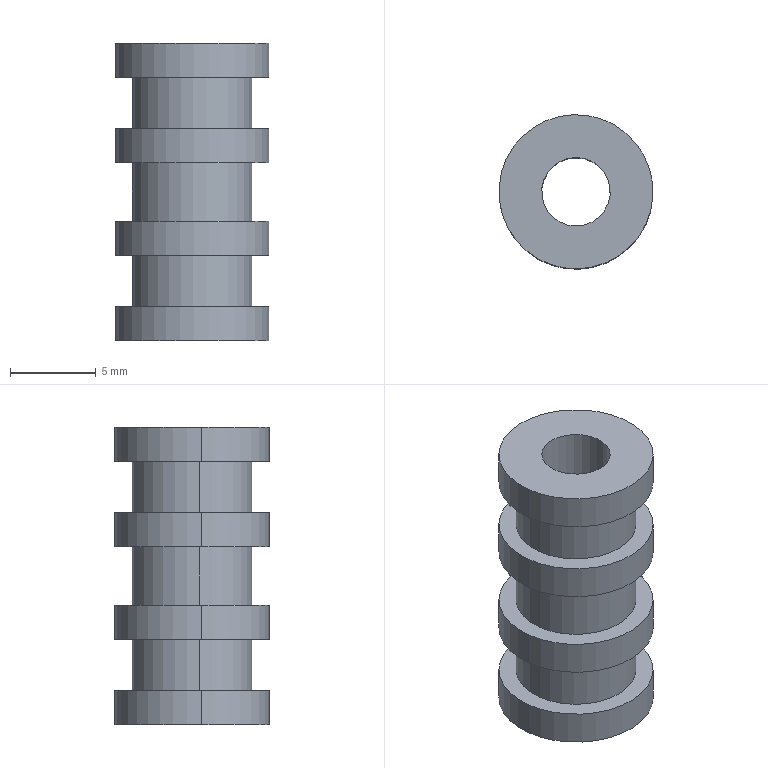Component | SolidWorks | TapeGuideRoller-1 | 1 solid | 24 faces | box 9 x 9 x 17.4 mm | volume 652 mm3 | cylinder 16 | plane 8 | commonest cylinder face diameters 9 x8 7 x6 4 x2
STEP:
#1=COLOUR_RGB('',0.7922,0.8196,0.9333);
#2=FILL_AREA_STYLE_COLOUR('',#1);
#3=FILL_AREA_STYLE('',(#2));
#4=SURFACE_STYLE_FILL_AREA(#3);
#5=SURFACE_SIDE_STYLE('',(#4));
#6=SURFACE_STYLE_USAGE(.BOTH.,#5);
#7=PRESENTATION_STYLE_ASSIGNMENT((#6));
#8=CARTESIAN_POINT('',(-6.397,4.985,1.713));
#9=VERTEX_POINT('',#8);
#10=CARTESIAN_POINT('',(-6.241,5.004,1.713));
#11=VERTEX_POINT('',#10);
#12=CARTESIAN_POINT('',(-6.319,4.995,1.713));
#13=DIRECTION('',(-0.,0.,-1.));
#14=DIRECTION('',(0.9922,0.1244,0.));
#15=AXIS2_PLACEMENT_3D('',#12,#13,#14);
#16=CIRCLE('',#15,0.07874);
#17=EDGE_CURVE('',#9,#11,#16,.T.);
#18=ORIENTED_EDGE('',*,*,#17,.F.);
#19=CARTESIAN_POINT('',(-6.397,4.985,1.028));
#20=VERTEX_POINT('',#19);
#21=CARTESIAN_POINT('',(-6.397,4.985,0.4858));
#22=DIRECTION('',(-0.,0.,-1.));
#23=VECTOR('',#22,39.37);
#24=LINE('',#21,#23);
#25=EDGE_CURVE('',#9,#20,#24,.T.);
#26=ORIENTED_EDGE('',*,*,#25,.T.);
#27=CARTESIAN_POINT('',(-6.241,5.004,1.028));
#28=VERTEX_POINT('',#27);
#29=CARTESIAN_POINT('',(-6.319,4.995,1.028));
#30=DIRECTION('',(0.,-0.,1.));
#31=DIRECTION('',(0.9922,0.1244,0.));
#32=AXIS2_PLACEMENT_3D('',#29,#30,#31);
#33=CIRCLE('',#32,0.07874);
#34=EDGE_CURVE('',#28,#20,#33,.T.);
#35=ORIENTED_EDGE('',*,*,#34,.F.);
#36=CARTESIAN_POINT('',(-6.241,5.004,0.4858));
#37=DIRECTION('',(-0.,0.,-1.));
#38=VECTOR('',#37,39.37);
#39=LINE('',#36,#38);
#40=EDGE_CURVE('',#11,#28,#39,.T.);
#41=ORIENTED_EDGE('',*,*,#40,.F.);
#42=EDGE_LOOP('',(#18,#26,#35,#41));
#43=FACE_OUTER_BOUND('',#42,.T.);
#44=CARTESIAN_POINT('',(-6.319,4.995,0.4858));
#45=DIRECTION('',(-0.,0.,-1.));
#46=DIRECTION('',(0.9922,0.1244,0.));
#47=AXIS2_PLACEMENT_3D('',#44,#45,#46);
#48=CYLINDRICAL_SURFACE('',#47,0.07874);
#49=ADVANCED_FACE('',(#43),#48,.F.);
#50=CARTESIAN_POINT('',(-6.143,5.017,1.713));
#51=VERTEX_POINT('',#50);
#52=CARTESIAN_POINT('',(-6.495,4.973,1.713));
#53=VERTEX_POINT('',#52);
#54=CARTESIAN_POINT('',(-6.319,4.995,1.713));
#55=DIRECTION('',(-0.,0.,-1.));
#56=DIRECTION('',(0.9922,0.1244,0.));
#57=AXIS2_PLACEMENT_3D('',#54,#55,#56);
#58=CIRCLE('',#57,0.1772);
#59=EDGE_CURVE('',#51,#53,#58,.T.);
#60=ORIENTED_EDGE('',*,*,#59,.T.);
#61=CARTESIAN_POINT('',(-6.495,4.973,1.634));
#62=VERTEX_POINT('',#61);
#63=CARTESIAN_POINT('',(-6.495,4.973,0.4858));
#64=DIRECTION('',(-0.,0.,-1.));
#65=VECTOR('',#64,39.37);
#66=LINE('',#63,#65);
#67=EDGE_CURVE('',#53,#62,#66,.T.);
#68=ORIENTED_EDGE('',*,*,#67,.T.);
#69=CARTESIAN_POINT('',(-6.143,5.017,1.634));
#70=VERTEX_POINT('',#69);
#71=CARTESIAN_POINT('',(-6.319,4.995,1.634));
#72=DIRECTION('',(0.,-0.,1.));
#73=DIRECTION('',(0.9922,0.1244,0.));
#74=AXIS2_PLACEMENT_3D('',#71,#72,#73);
#75=CIRCLE('',#74,0.1772);
#76=EDGE_CURVE('',#62,#70,#75,.T.);
#77=ORIENTED_EDGE('',*,*,#76,.T.);
#78=CARTESIAN_POINT('',(-6.143,5.017,0.4858));
#79=DIRECTION('',(-0.,0.,-1.));
#80=VECTOR('',#79,39.37);
#81=LINE('',#78,#80);
#82=EDGE_CURVE('',#51,#70,#81,.T.);
#83=ORIENTED_EDGE('',*,*,#82,.F.);
#84=EDGE_LOOP('',(#60,#68,#77,#83));
#85=FACE_OUTER_BOUND('',#84,.T.);
#86=CARTESIAN_POINT('',(-6.319,4.995,0.4858));
#87=DIRECTION('',(-0.,0.,-1.));
#88=DIRECTION('',(0.9922,0.1244,0.));
#89=AXIS2_PLACEMENT_3D('',#86,#87,#88);
#90=CYLINDRICAL_SURFACE('',#89,0.1772);
#91=ADVANCED_FACE('',(#85),#90,.T.);
#92=CARTESIAN_POINT('',(-6.143,5.017,1.106));
#93=VERTEX_POINT('',#92);
#94=CARTESIAN_POINT('',(-6.495,4.973,1.106));
#95=VERTEX_POINT('',#94);
#96=CARTESIAN_POINT('',(-6.319,4.995,1.106));
#97=DIRECTION('',(-0.,0.,-1.));
#98=DIRECTION('',(0.9922,0.1244,0.));
#99=AXIS2_PLACEMENT_3D('',#96,#97,#98);
#100=CIRCLE('',#99,0.1772);
#101=EDGE_CURVE('',#93,#95,#100,.T.);
#102=ORIENTED_EDGE('',*,*,#101,.T.);
#103=CARTESIAN_POINT('',(-6.495,4.973,1.028));
#104=VERTEX_POINT('',#103);
#105=CARTESIAN_POINT('',(-6.495,4.973,0.4858));
#106=DIRECTION('',(-0.,0.,-1.));
#107=VECTOR('',#106,39.37);
#108=LINE('',#105,#107);
#109=EDGE_CURVE('',#95,#104,#108,.T.);
#110=ORIENTED_EDGE('',*,*,#109,.T.);
#111=CARTESIAN_POINT('',(-6.143,5.017,1.028));
#112=VERTEX_POINT('',#111);
#113=CARTESIAN_POINT('',(-6.319,4.995,1.028));
#114=DIRECTION('',(0.,-0.,1.));
#115=DIRECTION('',(0.9922,0.1244,0.));
#116=AXIS2_PLACEMENT_3D('',#113,#114,#115);
#117=CIRCLE('',#116,0.1772);
#118=EDGE_CURVE('',#104,#112,#117,.T.);
#119=ORIENTED_EDGE('',*,*,#118,.T.);
#120=CARTESIAN_POINT('',(-6.143,5.017,0.4858));
#121=DIRECTION('',(-0.,0.,-1.));
#122=VECTOR('',#121,39.37);
#123=LINE('',#120,#122);
#124=EDGE_CURVE('',#93,#112,#123,.T.);
#125=ORIENTED_EDGE('',*,*,#124,.F.);
#126=EDGE_LOOP('',(#102,#110,#119,#125));
#127=FACE_OUTER_BOUND('',#126,.T.);
#128=CARTESIAN_POINT('',(-6.319,4.995,0.4858));
#129=DIRECTION('',(-0.,0.,-1.));
#130=DIRECTION('',(0.9922,0.1244,0.));
#131=AXIS2_PLACEMENT_3D('',#128,#129,#130);
#132=CYLINDRICAL_SURFACE('',#131,0.1772);
#133=ADVANCED_FACE('',(#127),#132,.T.);
#134=CARTESIAN_POINT('',(-6.182,5.012,1.634));
#135=VERTEX_POINT('',#134);
#136=CARTESIAN_POINT('',(-6.456,4.978,1.634));
#137=VERTEX_POINT('',#136);
#138=CARTESIAN_POINT('',(-6.319,4.995,1.634));
#139=DIRECTION('',(-0.,0.,-1.));
#140=DIRECTION('',(0.9922,0.1244,0.));
#141=AXIS2_PLACEMENT_3D('',#138,#139,#140);
#142=CIRCLE('',#141,0.1378);
#143=EDGE_CURVE('',#135,#137,#142,.T.);
#144=ORIENTED_EDGE('',*,*,#143,.T.);
#145=CARTESIAN_POINT('',(-6.456,4.978,1.516));
#146=VERTEX_POINT('',#145);
#147=CARTESIAN_POINT('',(-6.456,4.978,0.4858));
#148=DIRECTION('',(-0.,0.,-1.));
#149=VECTOR('',#148,39.37);
#150=LINE('',#147,#149);
#151=EDGE_CURVE('',#137,#146,#150,.T.);
#152=ORIENTED_EDGE('',*,*,#151,.T.);
#153=CARTESIAN_POINT('',(-6.182,5.012,1.516));
#154=VERTEX_POINT('',#153);
#155=CARTESIAN_POINT('',(-6.319,4.995,1.516));
#156=DIRECTION('',(0.,-0.,1.));
#157=DIRECTION('',(0.9922,0.1244,0.));
#158=AXIS2_PLACEMENT_3D('',#155,#156,#157);
#159=CIRCLE('',#158,0.1378);
#160=EDGE_CURVE('',#146,#154,#159,.T.);
#161=ORIENTED_EDGE('',*,*,#160,.T.);
#162=CARTESIAN_POINT('',(-6.182,5.012,0.4858));
#163=DIRECTION('',(-0.,0.,-1.));
#164=VECTOR('',#163,39.37);
#165=LINE('',#162,#164);
#166=EDGE_CURVE('',#135,#154,#165,.T.);
#167=ORIENTED_EDGE('',*,*,#166,.F.);
#168=EDGE_LOOP('',(#144,#152,#161,#167));
#169=FACE_OUTER_BOUND('',#168,.T.);
#170=CARTESIAN_POINT('',(-6.319,4.995,0.4858));
#171=DIRECTION('',(-0.,0.,-1.));
#172=DIRECTION('',(0.9922,0.1244,0.));
#173=AXIS2_PLACEMENT_3D('',#170,#171,#172);
#174=CYLINDRICAL_SURFACE('',#173,0.1378);
#175=ADVANCED_FACE('',(#169),#174,.T.);
#176=CARTESIAN_POINT('',(-6.182,5.012,1.224));
#177=VERTEX_POINT('',#176);
#178=CARTESIAN_POINT('',(-6.456,4.978,1.224));
#179=VERTEX_POINT('',#178);
#180=CARTESIAN_POINT('',(-6.319,4.995,1.224));
#181=DIRECTION('',(-0.,0.,-1.));
#182=DIRECTION('',(0.9922,0.1244,0.));
#183=AXIS2_PLACEMENT_3D('',#180,#181,#182);
#184=CIRCLE('',#183,0.1378);
#185=EDGE_CURVE('',#177,#179,#184,.T.);
#186=ORIENTED_EDGE('',*,*,#185,.T.);
#187=CARTESIAN_POINT('',(-6.456,4.978,1.106));
#188=VERTEX_POINT('',#187);
#189=CARTESIAN_POINT('',(-6.456,4.978,0.4858));
#190=DIRECTION('',(-0.,0.,-1.));
#191=VECTOR('',#190,39.37);
#192=LINE('',#189,#191);
#193=EDGE_CURVE('',#179,#188,#192,.T.);
#194=ORIENTED_EDGE('',*,*,#193,.T.);
#195=CARTESIAN_POINT('',(-6.182,5.012,1.106));
#196=VERTEX_POINT('',#195);
#197=CARTESIAN_POINT('',(-6.319,4.995,1.106));
#198=DIRECTION('',(0.,-0.,1.));
#199=DIRECTION('',(0.9922,0.1244,0.));
#200=AXIS2_PLACEMENT_3D('',#197,#198,#199);
#201=CIRCLE('',#200,0.1378);
#202=EDGE_CURVE('',#188,#196,#201,.T.);
#203=ORIENTED_EDGE('',*,*,#202,.T.);
#204=CARTESIAN_POINT('',(-6.182,5.012,0.4858));
#205=DIRECTION('',(-0.,0.,-1.));
#206=VECTOR('',#205,39.37);
#207=LINE('',#204,#206);
#208=EDGE_CURVE('',#177,#196,#207,.T.);
#209=ORIENTED_EDGE('',*,*,#208,.F.);
#210=EDGE_LOOP('',(#186,#194,#203,#209));
#211=FACE_OUTER_BOUND('',#210,.T.);
#212=CARTESIAN_POINT('',(-6.319,4.995,0.4858));
#213=DIRECTION('',(-0.,0.,-1.));
#214=DIRECTION('',(0.9922,0.1244,0.));
#215=AXIS2_PLACEMENT_3D('',#212,#213,#214);
#216=CYLINDRICAL_SURFACE('',#215,0.1378);
#217=ADVANCED_FACE('',(#211),#216,.T.);
#218=CARTESIAN_POINT('',(-6.143,5.017,1.516));
#219=VERTEX_POINT('',#218);
#220=CARTESIAN_POINT('',(-6.495,4.973,1.516));
#221=VERTEX_POINT('',#220);
#222=CARTESIAN_POINT('',(-6.319,4.995,1.516));
#223=DIRECTION('',(-0.,0.,-1.));
#224=DIRECTION('',(0.9922,0.1244,0.));
#225=AXIS2_PLACEMENT_3D('',#222,#223,#224);
#226=CIRCLE('',#225,0.1772);
#227=EDGE_CURVE('',#219,#221,#226,.T.);
#228=ORIENTED_EDGE('',*,*,#227,.T.);
#229=CARTESIAN_POINT('',(-6.495,4.973,1.437));
#230=VERTEX_POINT('',#229);
#231=CARTESIAN_POINT('',(-6.495,4.973,0.4858));
#232=DIRECTION('',(-0.,0.,-1.));
#233=VECTOR('',#232,39.37);
#234=LINE('',#231,#233);
#235=EDGE_CURVE('',#221,#230,#234,.T.);
#236=ORIENTED_EDGE('',*,*,#235,.T.);
#237=CARTESIAN_POINT('',(-6.143,5.017,1.437));
#238=VERTEX_POINT('',#237);
#239=CARTESIAN_POINT('',(-6.319,4.995,1.437));
#240=DIRECTION('',(0.,-0.,1.));
#241=DIRECTION('',(0.9922,0.1244,0.));
#242=AXIS2_PLACEMENT_3D('',#239,#240,#241);
#243=CIRCLE('',#242,0.1772);
#244=EDGE_CURVE('',#230,#238,#243,.T.);
#245=ORIENTED_EDGE('',*,*,#244,.T.);
#246=CARTESIAN_POINT('',(-6.143,5.017,0.4858));
#247=DIRECTION('',(-0.,0.,-1.));
#248=VECTOR('',#247,39.37);
#249=LINE('',#246,#248);
#250=EDGE_CURVE('',#219,#238,#249,.T.);
#251=ORIENTED_EDGE('',*,*,#250,.F.);
#252=EDGE_LOOP('',(#228,#236,#245,#251));
#253=FACE_OUTER_BOUND('',#252,.T.);
#254=CARTESIAN_POINT('',(-6.319,4.995,0.4858));
#255=DIRECTION('',(-0.,0.,-1.));
#256=DIRECTION('',(0.9922,0.1244,0.));
#257=AXIS2_PLACEMENT_3D('',#254,#255,#256);
#258=CYLINDRICAL_SURFACE('',#257,0.1772);
#259=ADVANCED_FACE('',(#253),#258,.T.);
#260=CARTESIAN_POINT('',(-6.143,5.017,1.303));
#261=VERTEX_POINT('',#260);
#262=CARTESIAN_POINT('',(-6.495,4.973,1.303));
#263=VERTEX_POINT('',#262);
#264=CARTESIAN_POINT('',(-6.319,4.995,1.303));
#265=DIRECTION('',(-0.,0.,-1.));
#266=DIRECTION('',(0.9922,0.1244,0.));
#267=AXIS2_PLACEMENT_3D('',#264,#265,#266);
#268=CIRCLE('',#267,0.1772);
#269=EDGE_CURVE('',#261,#263,#268,.T.);
#270=ORIENTED_EDGE('',*,*,#269,.T.);
#271=CARTESIAN_POINT('',(-6.495,4.973,1.224));
#272=VERTEX_POINT('',#271);
#273=CARTESIAN_POINT('',(-6.495,4.973,0.4858));
#274=DIRECTION('',(-0.,0.,-1.));
#275=VECTOR('',#274,39.37);
#276=LINE('',#273,#275);
#277=EDGE_CURVE('',#263,#272,#276,.T.);
#278=ORIENTED_EDGE('',*,*,#277,.T.);
#279=CARTESIAN_POINT('',(-6.143,5.017,1.224));
#280=VERTEX_POINT('',#279);
#281=CARTESIAN_POINT('',(-6.319,4.995,1.224));
#282=DIRECTION('',(0.,-0.,1.));
#283=DIRECTION('',(0.9922,0.1244,0.));
#284=AXIS2_PLACEMENT_3D('',#281,#282,#283);
#285=CIRCLE('',#284,0.1772);
#286=EDGE_CURVE('',#272,#280,#285,.T.);
#287=ORIENTED_EDGE('',*,*,#286,.T.);
#288=CARTESIAN_POINT('',(-6.143,5.017,0.4858));
#289=DIRECTION('',(-0.,0.,-1.));
#290=VECTOR('',#289,39.37);
#291=LINE('',#288,#290);
#292=EDGE_CURVE('',#261,#280,#291,.T.);
#293=ORIENTED_EDGE('',*,*,#292,.F.);
#294=EDGE_LOOP('',(#270,#278,#287,#293));
#295=FACE_OUTER_BOUND('',#294,.T.);
#296=CARTESIAN_POINT('',(-6.319,4.995,0.4858));
#297=DIRECTION('',(-0.,0.,-1.));
#298=DIRECTION('',(0.9922,0.1244,0.));
#299=AXIS2_PLACEMENT_3D('',#296,#297,#298);
#300=CYLINDRICAL_SURFACE('',#299,0.1772);
#301=ADVANCED_FACE('',(#295),#300,.T.);
#302=CARTESIAN_POINT('',(-6.182,5.012,1.437));
#303=VERTEX_POINT('',#302);
#304=CARTESIAN_POINT('',(-6.456,4.978,1.437));
#305=VERTEX_POINT('',#304);
#306=CARTESIAN_POINT('',(-6.319,4.995,1.437));
#307=DIRECTION('',(-0.,0.,-1.));
#308=DIRECTION('',(0.9922,0.1244,0.));
#309=AXIS2_PLACEMENT_3D('',#306,#307,#308);
#310=CIRCLE('',#309,0.1378);
#311=EDGE_CURVE('',#303,#305,#310,.T.);
#312=ORIENTED_EDGE('',*,*,#311,.T.);
#313=CARTESIAN_POINT('',(-6.456,4.978,1.303));
#314=VERTEX_POINT('',#313);
#315=CARTESIAN_POINT('',(-6.456,4.978,0.4858));
#316=DIRECTION('',(-0.,0.,-1.));
#317=VECTOR('',#316,39.37);
#318=LINE('',#315,#317);
#319=EDGE_CURVE('',#305,#314,#318,.T.);
#320=ORIENTED_EDGE('',*,*,#319,.T.);
#321=CARTESIAN_POINT('',(-6.182,5.012,1.303));
#322=VERTEX_POINT('',#321);
#323=CARTESIAN_POINT('',(-6.319,4.995,1.303));
#324=DIRECTION('',(0.,-0.,1.));
#325=DIRECTION('',(0.9922,0.1244,0.));
#326=AXIS2_PLACEMENT_3D('',#323,#324,#325);
#327=CIRCLE('',#326,0.1378);
#328=EDGE_CURVE('',#314,#322,#327,.T.);
#329=ORIENTED_EDGE('',*,*,#328,.T.);
#330=CARTESIAN_POINT('',(-6.182,5.012,0.4858));
#331=DIRECTION('',(-0.,0.,-1.));
#332=VECTOR('',#331,39.37);
#333=LINE('',#330,#332);
#334=EDGE_CURVE('',#303,#322,#333,.T.);
#335=ORIENTED_EDGE('',*,*,#334,.F.);
#336=EDGE_LOOP('',(#312,#320,#329,#335));
#337=FACE_OUTER_BOUND('',#336,.T.);
#338=CARTESIAN_POINT('',(-6.319,4.995,0.4858));
#339=DIRECTION('',(-0.,0.,-1.));
#340=DIRECTION('',(0.9922,0.1244,0.));
#341=AXIS2_PLACEMENT_3D('',#338,#339,#340);
#342=CYLINDRICAL_SURFACE('',#341,0.1378);
#343=ADVANCED_FACE('',(#337),#342,.T.);
#344=ORIENTED_EDGE('',*,*,#25,.F.);
#345=CARTESIAN_POINT('',(-6.319,4.995,1.713));
#346=DIRECTION('',(-0.,0.,-1.));
#347=DIRECTION('',(0.9922,0.1244,0.));
#348=AXIS2_PLACEMENT_3D('',#345,#346,#347);
#349=CIRCLE('',#348,0.07874);
#350=EDGE_CURVE('',#11,#9,#349,.T.);
#351=ORIENTED_EDGE('',*,*,#350,.F.);
#352=ORIENTED_EDGE('',*,*,#40,.T.);
#353=CARTESIAN_POINT('',(-6.319,4.995,1.028));
#354=DIRECTION('',(0.,-0.,1.));
#355=DIRECTION('',(0.9922,0.1244,0.));
#356=AXIS2_PLACEMENT_3D('',#353,#354,#355);
#357=CIRCLE('',#356,0.07874);
#358=EDGE_CURVE('',#20,#28,#357,.T.);
#359=ORIENTED_EDGE('',*,*,#358,.F.);
#360=EDGE_LOOP('',(#344,#351,#352,#359));
#361=FACE_OUTER_BOUND('',#360,.T.);
#362=CARTESIAN_POINT('',(-6.319,4.995,0.4858));
#363=DIRECTION('',(-0.,0.,-1.));
#364=DIRECTION('',(0.9922,0.1244,0.));
#365=AXIS2_PLACEMENT_3D('',#362,#363,#364);
#366=CYLINDRICAL_SURFACE('',#365,0.07874);
#367=ADVANCED_FACE('',(#361),#366,.F.);
#368=ORIENTED_EDGE('',*,*,#350,.T.);
#369=ORIENTED_EDGE('',*,*,#17,.T.);
#370=EDGE_LOOP('',(#368,#369));
#371=FACE_BOUND('',#370,.T.);
#372=ORIENTED_EDGE('',*,*,#59,.F.);
#373=CARTESIAN_POINT('',(-6.319,4.995,1.713));
#374=DIRECTION('',(-0.,0.,-1.));
#375=DIRECTION('',(0.9922,0.1244,0.));
#376=AXIS2_PLACEMENT_3D('',#373,#374,#375);
#377=CIRCLE('',#376,0.1772);
#378=EDGE_CURVE('',#53,#51,#377,.T.);
#379=ORIENTED_EDGE('',*,*,#378,.F.);
#380=EDGE_LOOP('',(#372,#379));
#381=FACE_OUTER_BOUND('',#380,.T.);
#382=CARTESIAN_POINT('',(-6.297,4.819,1.713));
#383=DIRECTION('',(-0.,0.,-1.));
#384=DIRECTION('',(0.9922,0.1244,0.));
#385=AXIS2_PLACEMENT_3D('',#382,#383,#384);
#386=PLANE('',#385);
#387=ADVANCED_FACE('',(#371,#381),#386,.F.);
#388=CARTESIAN_POINT('',(-6.319,4.995,1.028));
#389=DIRECTION('',(0.,-0.,1.));
#390=DIRECTION('',(0.9922,0.1244,0.));
#391=AXIS2_PLACEMENT_3D('',#388,#389,#390);
#392=CIRCLE('',#391,0.1772);
#393=EDGE_CURVE('',#112,#104,#392,.T.);
#394=ORIENTED_EDGE('',*,*,#393,.F.);
#395=ORIENTED_EDGE('',*,*,#118,.F.);
#396=EDGE_LOOP('',(#394,#395));
#397=FACE_OUTER_BOUND('',#396,.T.);
#398=ORIENTED_EDGE('',*,*,#34,.T.);
#399=ORIENTED_EDGE('',*,*,#358,.T.);
#400=EDGE_LOOP('',(#398,#399));
#401=FACE_BOUND('',#400,.T.);
#402=CARTESIAN_POINT('',(-6.297,4.819,1.028));
#403=DIRECTION('',(0.,-0.,1.));
#404=DIRECTION('',(-0.9922,-0.1244,-0.));
#405=AXIS2_PLACEMENT_3D('',#402,#403,#404);
#406=PLANE('',#405);
#407=ADVANCED_FACE('',(#397,#401),#406,.F.);
#408=ORIENTED_EDGE('',*,*,#67,.F.);
#409=ORIENTED_EDGE('',*,*,#378,.T.);
#410=ORIENTED_EDGE('',*,*,#82,.T.);
#411=CARTESIAN_POINT('',(-6.319,4.995,1.634));
#412=DIRECTION('',(0.,-0.,1.));
#413=DIRECTION('',(0.9922,0.1244,0.));
#414=AXIS2_PLACEMENT_3D('',#411,#412,#413);
#415=CIRCLE('',#414,0.1772);
#416=EDGE_CURVE('',#70,#62,#415,.T.);
#417=ORIENTED_EDGE('',*,*,#416,.T.);
#418=EDGE_LOOP('',(#408,#409,#410,#417));
#419=FACE_OUTER_BOUND('',#418,.T.);
#420=CARTESIAN_POINT('',(-6.319,4.995,0.4858));
#421=DIRECTION('',(-0.,0.,-1.));
#422=DIRECTION('',(0.9922,0.1244,0.));
#423=AXIS2_PLACEMENT_3D('',#420,#421,#422);
#424=CYLINDRICAL_SURFACE('',#423,0.1772);
#425=ADVANCED_FACE('',(#419),#424,.T.);
#426=ORIENTED_EDGE('',*,*,#109,.F.);
#427=CARTESIAN_POINT('',(-6.319,4.995,1.106));
#428=DIRECTION('',(-0.,0.,-1.));
#429=DIRECTION('',(0.9922,0.1244,0.));
#430=AXIS2_PLACEMENT_3D('',#427,#428,#429);
#431=CIRCLE('',#430,0.1772);
#432=EDGE_CURVE('',#95,#93,#431,.T.);
#433=ORIENTED_EDGE('',*,*,#432,.T.);
#434=ORIENTED_EDGE('',*,*,#124,.T.);
#435=ORIENTED_EDGE('',*,*,#393,.T.);
#436=EDGE_LOOP('',(#426,#433,#434,#435));
#437=FACE_OUTER_BOUND('',#436,.T.);
#438=CARTESIAN_POINT('',(-6.319,4.995,0.4858));
#439=DIRECTION('',(-0.,0.,-1.));
#440=DIRECTION('',(0.9922,0.1244,0.));
#441=AXIS2_PLACEMENT_3D('',#438,#439,#440);
#442=CYLINDRICAL_SURFACE('',#441,0.1772);
#443=ADVANCED_FACE('',(#437),#442,.T.);
#444=ORIENTED_EDGE('',*,*,#416,.F.);
#445=ORIENTED_EDGE('',*,*,#76,.F.);
#446=EDGE_LOOP('',(#444,#445));
#447=FACE_OUTER_BOUND('',#446,.T.);
#448=ORIENTED_EDGE('',*,*,#143,.F.);
#449=CARTESIAN_POINT('',(-6.319,4.995,1.634));
#450=DIRECTION('',(-0.,0.,-1.));
#451=DIRECTION('',(0.9922,0.1244,0.));
#452=AXIS2_PLACEMENT_3D('',#449,#450,#451);
#453=CIRCLE('',#452,0.1378);
#454=EDGE_CURVE('',#137,#135,#453,.T.);
#455=ORIENTED_EDGE('',*,*,#454,.F.);
#456=EDGE_LOOP('',(#448,#455));
#457=FACE_BOUND('',#456,.T.);
#458=CARTESIAN_POINT('',(-6.302,4.858,1.634));
#459=DIRECTION('',(0.,-0.,1.));
#460=DIRECTION('',(-0.9922,-0.1244,-0.));
#461=AXIS2_PLACEMENT_3D('',#458,#459,#460);
#462=PLANE('',#461);
#463=ADVANCED_FACE('',(#447,#457),#462,.F.);
#464=CARTESIAN_POINT('',(-6.319,4.995,1.106));
#465=DIRECTION('',(0.,-0.,1.));
#466=DIRECTION('',(0.9922,0.1244,0.));
#467=AXIS2_PLACEMENT_3D('',#464,#465,#466);
#468=CIRCLE('',#467,0.1378);
#469=EDGE_CURVE('',#196,#188,#468,.T.);
#470=ORIENTED_EDGE('',*,*,#469,.F.);
#471=ORIENTED_EDGE('',*,*,#202,.F.);
#472=EDGE_LOOP('',(#470,#471));
#473=FACE_BOUND('',#472,.T.);
#474=ORIENTED_EDGE('',*,*,#101,.F.);
#475=ORIENTED_EDGE('',*,*,#432,.F.);
#476=EDGE_LOOP('',(#474,#475));
#477=FACE_OUTER_BOUND('',#476,.T.);
#478=CARTESIAN_POINT('',(-6.297,4.819,1.106));
#479=DIRECTION('',(-0.,0.,-1.));
#480=DIRECTION('',(0.9922,0.1244,0.));
#481=AXIS2_PLACEMENT_3D('',#478,#479,#480);
#482=PLANE('',#481);
#483=ADVANCED_FACE('',(#473,#477),#482,.F.);
#484=ORIENTED_EDGE('',*,*,#151,.F.);
#485=ORIENTED_EDGE('',*,*,#454,.T.);
#486=ORIENTED_EDGE('',*,*,#166,.T.);
#487=CARTESIAN_POINT('',(-6.319,4.995,1.516));
#488=DIRECTION('',(0.,-0.,1.));
#489=DIRECTION('',(0.9922,0.1244,0.));
#490=AXIS2_PLACEMENT_3D('',#487,#488,#489);
#491=CIRCLE('',#490,0.1378);
#492=EDGE_CURVE('',#154,#146,#491,.T.);
#493=ORIENTED_EDGE('',*,*,#492,.T.);
#494=EDGE_LOOP('',(#484,#485,#486,#493));
#495=FACE_OUTER_BOUND('',#494,.T.);
#496=CARTESIAN_POINT('',(-6.319,4.995,0.4858));
#497=DIRECTION('',(-0.,0.,-1.));
#498=DIRECTION('',(0.9922,0.1244,0.));
#499=AXIS2_PLACEMENT_3D('',#496,#497,#498);
#500=CYLINDRICAL_SURFACE('',#499,0.1378);
#501=ADVANCED_FACE('',(#495),#500,.T.);
#502=ORIENTED_EDGE('',*,*,#193,.F.);
#503=CARTESIAN_POINT('',(-6.319,4.995,1.224));
#504=DIRECTION('',(-0.,0.,-1.));
#505=DIRECTION('',(0.9922,0.1244,0.));
#506=AXIS2_PLACEMENT_3D('',#503,#504,#505);
#507=CIRCLE('',#506,0.1378);
#508=EDGE_CURVE('',#179,#177,#507,.T.);
#509=ORIENTED_EDGE('',*,*,#508,.T.);
#510=ORIENTED_EDGE('',*,*,#208,.T.);
#511=ORIENTED_EDGE('',*,*,#469,.T.);
#512=EDGE_LOOP('',(#502,#509,#510,#511));
#513=FACE_OUTER_BOUND('',#512,.T.);
#514=CARTESIAN_POINT('',(-6.319,4.995,0.4858));
#515=DIRECTION('',(-0.,0.,-1.));
#516=DIRECTION('',(0.9922,0.1244,0.));
#517=AXIS2_PLACEMENT_3D('',#514,#515,#516);
#518=CYLINDRICAL_SURFACE('',#517,0.1378);
#519=ADVANCED_FACE('',(#513),#518,.T.);
#520=ORIENTED_EDGE('',*,*,#492,.F.);
#521=ORIENTED_EDGE('',*,*,#160,.F.);
#522=EDGE_LOOP('',(#520,#521));
#523=FACE_BOUND('',#522,.T.);
#524=ORIENTED_EDGE('',*,*,#227,.F.);
#525=CARTESIAN_POINT('',(-6.319,4.995,1.516));
#526=DIRECTION('',(-0.,0.,-1.));
#527=DIRECTION('',(0.9922,0.1244,0.));
#528=AXIS2_PLACEMENT_3D('',#525,#526,#527);
#529=CIRCLE('',#528,0.1772);
#530=EDGE_CURVE('',#221,#219,#529,.T.);
#531=ORIENTED_EDGE('',*,*,#530,.F.);
#532=EDGE_LOOP('',(#524,#531));
#533=FACE_OUTER_BOUND('',#532,.T.);
#534=CARTESIAN_POINT('',(-6.297,4.819,1.516));
#535=DIRECTION('',(-0.,0.,-1.));
#536=DIRECTION('',(0.9922,0.1244,0.));
#537=AXIS2_PLACEMENT_3D('',#534,#535,#536);
#538=PLANE('',#537);
#539=ADVANCED_FACE('',(#523,#533),#538,.F.);
#540=CARTESIAN_POINT('',(-6.319,4.995,1.224));
#541=DIRECTION('',(0.,-0.,1.));
#542=DIRECTION('',(0.9922,0.1244,0.));
#543=AXIS2_PLACEMENT_3D('',#540,#541,#542);
#544=CIRCLE('',#543,0.1772);
#545=EDGE_CURVE('',#280,#272,#544,.T.);
#546=ORIENTED_EDGE('',*,*,#545,.F.);
#547=ORIENTED_EDGE('',*,*,#286,.F.);
#548=EDGE_LOOP('',(#546,#547));
#549=FACE_OUTER_BOUND('',#548,.T.);
#550=ORIENTED_EDGE('',*,*,#185,.F.);
#551=ORIENTED_EDGE('',*,*,#508,.F.);
#552=EDGE_LOOP('',(#550,#551));
#553=FACE_BOUND('',#552,.T.);
#554=CARTESIAN_POINT('',(-6.302,4.858,1.224));
#555=DIRECTION('',(0.,-0.,1.));
#556=DIRECTION('',(-0.9922,-0.1244,-0.));
#557=AXIS2_PLACEMENT_3D('',#554,#555,#556);
#558=PLANE('',#557);
#559=ADVANCED_FACE('',(#549,#553),#558,.F.);
#560=ORIENTED_EDGE('',*,*,#235,.F.);
#561=ORIENTED_EDGE('',*,*,#530,.T.);
#562=ORIENTED_EDGE('',*,*,#250,.T.);
#563=CARTESIAN_POINT('',(-6.319,4.995,1.437));
#564=DIRECTION('',(0.,-0.,1.));
#565=DIRECTION('',(0.9922,0.1244,0.));
#566=AXIS2_PLACEMENT_3D('',#563,#564,#565);
#567=CIRCLE('',#566,0.1772);
#568=EDGE_CURVE('',#238,#230,#567,.T.);
#569=ORIENTED_EDGE('',*,*,#568,.T.);
#570=EDGE_LOOP('',(#560,#561,#562,#569));
#571=FACE_OUTER_BOUND('',#570,.T.);
#572=CARTESIAN_POINT('',(-6.319,4.995,0.4858));
#573=DIRECTION('',(-0.,0.,-1.));
#574=DIRECTION('',(0.9922,0.1244,0.));
#575=AXIS2_PLACEMENT_3D('',#572,#573,#574);
#576=CYLINDRICAL_SURFACE('',#575,0.1772);
#577=ADVANCED_FACE('',(#571),#576,.T.);
#578=ORIENTED_EDGE('',*,*,#277,.F.);
#579=CARTESIAN_POINT('',(-6.319,4.995,1.303));
#580=DIRECTION('',(-0.,0.,-1.));
#581=DIRECTION('',(0.9922,0.1244,0.));
#582=AXIS2_PLACEMENT_3D('',#579,#580,#581);
#583=CIRCLE('',#582,0.1772);
#584=EDGE_CURVE('',#263,#261,#583,.T.);
#585=ORIENTED_EDGE('',*,*,#584,.T.);
#586=ORIENTED_EDGE('',*,*,#292,.T.);
#587=ORIENTED_EDGE('',*,*,#545,.T.);
#588=EDGE_LOOP('',(#578,#585,#586,#587));
#589=FACE_OUTER_BOUND('',#588,.T.);
#590=CARTESIAN_POINT('',(-6.319,4.995,0.4858));
#591=DIRECTION('',(-0.,0.,-1.));
#592=DIRECTION('',(0.9922,0.1244,0.));
#593=AXIS2_PLACEMENT_3D('',#590,#591,#592);
#594=CYLINDRICAL_SURFACE('',#593,0.1772);
#595=ADVANCED_FACE('',(#589),#594,.T.);
#596=ORIENTED_EDGE('',*,*,#568,.F.);
#597=ORIENTED_EDGE('',*,*,#244,.F.);
#598=EDGE_LOOP('',(#596,#597));
#599=FACE_OUTER_BOUND('',#598,.T.);
#600=ORIENTED_EDGE('',*,*,#311,.F.);
#601=CARTESIAN_POINT('',(-6.319,4.995,1.437));
#602=DIRECTION('',(-0.,0.,-1.));
#603=DIRECTION('',(0.9922,0.1244,0.));
#604=AXIS2_PLACEMENT_3D('',#601,#602,#603);
#605=CIRCLE('',#604,0.1378);
#606=EDGE_CURVE('',#305,#303,#605,.T.);
#607=ORIENTED_EDGE('',*,*,#606,.F.);
#608=EDGE_LOOP('',(#600,#607));
#609=FACE_BOUND('',#608,.T.);
#610=CARTESIAN_POINT('',(-6.302,4.858,1.437));
#611=DIRECTION('',(0.,-0.,1.));
#612=DIRECTION('',(-0.9922,-0.1244,-0.));
#613=AXIS2_PLACEMENT_3D('',#610,#611,#612);
#614=PLANE('',#613);
#615=ADVANCED_FACE('',(#599,#609),#614,.F.);
#616=CARTESIAN_POINT('',(-6.319,4.995,1.303));
#617=DIRECTION('',(0.,-0.,1.));
#618=DIRECTION('',(0.9922,0.1244,0.));
#619=AXIS2_PLACEMENT_3D('',#616,#617,#618);
#620=CIRCLE('',#619,0.1378);
#621=EDGE_CURVE('',#322,#314,#620,.T.);
#622=ORIENTED_EDGE('',*,*,#621,.F.);
#623=ORIENTED_EDGE('',*,*,#328,.F.);
#624=EDGE_LOOP('',(#622,#623));
#625=FACE_BOUND('',#624,.T.);
#626=ORIENTED_EDGE('',*,*,#269,.F.);
#627=ORIENTED_EDGE('',*,*,#584,.F.);
#628=EDGE_LOOP('',(#626,#627));
#629=FACE_OUTER_BOUND('',#628,.T.);
#630=CARTESIAN_POINT('',(-6.297,4.819,1.303));
#631=DIRECTION('',(-0.,0.,-1.));
#632=DIRECTION('',(0.9922,0.1244,0.));
#633=AXIS2_PLACEMENT_3D('',#630,#631,#632);
#634=PLANE('',#633);
#635=ADVANCED_FACE('',(#625,#629),#634,.F.);
#636=ORIENTED_EDGE('',*,*,#319,.F.);
#637=ORIENTED_EDGE('',*,*,#606,.T.);
#638=ORIENTED_EDGE('',*,*,#334,.T.);
#639=ORIENTED_EDGE('',*,*,#621,.T.);
#640=EDGE_LOOP('',(#636,#637,#638,#639));
#641=FACE_OUTER_BOUND('',#640,.T.);
#642=CARTESIAN_POINT('',(-6.319,4.995,0.4858));
#643=DIRECTION('',(-0.,0.,-1.));
#644=DIRECTION('',(0.9922,0.1244,0.));
#645=AXIS2_PLACEMENT_3D('',#642,#643,#644);
#646=CYLINDRICAL_SURFACE('',#645,0.1378);
#647=ADVANCED_FACE('',(#641),#646,.T.);
#648=CLOSED_SHELL('',(#49,#91,#133,#175,#217,#259,#301,#343,#367,#387,#407,#425,#443,#463,#483,#501,#519,#539,#559,#577,#595,#615,#635,#647));
#649=MANIFOLD_SOLID_BREP('',#648);
#650=STYLED_ITEM('',(#7),#649);
#651=PRESENTATION_LAYER_ASSIGNMENT('','',(#650));
#652=CARTESIAN_POINT('',(0.,0.,0.));
#653=DIRECTION('',(0.,0.,1.));
#654=DIRECTION('',(1.,0.,0.));
#655=AXIS2_PLACEMENT_3D('',#652,#653,#654);
#656=(LENGTH_UNIT()NAMED_UNIT(*)SI_UNIT($,.METRE.));
#657=LENGTH_MEASURE_WITH_UNIT(LENGTH_MEASURE(0.0254),#656);
#658=DIMENSIONAL_EXPONENTS(1.,0.,0.,0.,0.,0.,0.);
#659=(CONVERSION_BASED_UNIT('',#657)LENGTH_UNIT()NAMED_UNIT(#658));
#660=UNCERTAINTY_MEASURE_WITH_UNIT(LENGTH_MEASURE(0.00001),#659,'','');
#661=(NAMED_UNIT(*)PLANE_ANGLE_UNIT()SI_UNIT($,.RADIAN.));
#662=(NAMED_UNIT(*)SI_UNIT($,.STERADIAN.)SOLID_ANGLE_UNIT());
#663=(GEOMETRIC_REPRESENTATION_CONTEXT(3)GLOBAL_UNCERTAINTY_ASSIGNED_CONTEXT((#660))GLOBAL_UNIT_ASSIGNED_CONTEXT((#659,#661,#662))REPRESENTATION_CONTEXT('',''));
#664=ADVANCED_BREP_SHAPE_REPRESENTATION('',(#649,#655),#663);
#665=(LENGTH_UNIT()NAMED_UNIT(*)SI_UNIT($,.METRE.));
#666=LENGTH_MEASURE_WITH_UNIT(LENGTH_MEASURE(0.0254),#665);
#667=DIMENSIONAL_EXPONENTS(1.,0.,0.,0.,0.,0.,0.);
#668=(CONVERSION_BASED_UNIT('',#666)LENGTH_UNIT()NAMED_UNIT(#667));
#669=UNCERTAINTY_MEASURE_WITH_UNIT(LENGTH_MEASURE(0.00001),#668,'','');
#670=(NAMED_UNIT(*)PLANE_ANGLE_UNIT()SI_UNIT($,.RADIAN.));
#671=(NAMED_UNIT(*)SI_UNIT($,.STERADIAN.)SOLID_ANGLE_UNIT());
#672=(GEOMETRIC_REPRESENTATION_CONTEXT(3)GLOBAL_UNCERTAINTY_ASSIGNED_CONTEXT((#669))GLOBAL_UNIT_ASSIGNED_CONTEXT((#668,#670,#671))REPRESENTATION_CONTEXT('',''));
#673=MECHANICAL_DESIGN_GEOMETRIC_PRESENTATION_REPRESENTATION('',(#650),#672);